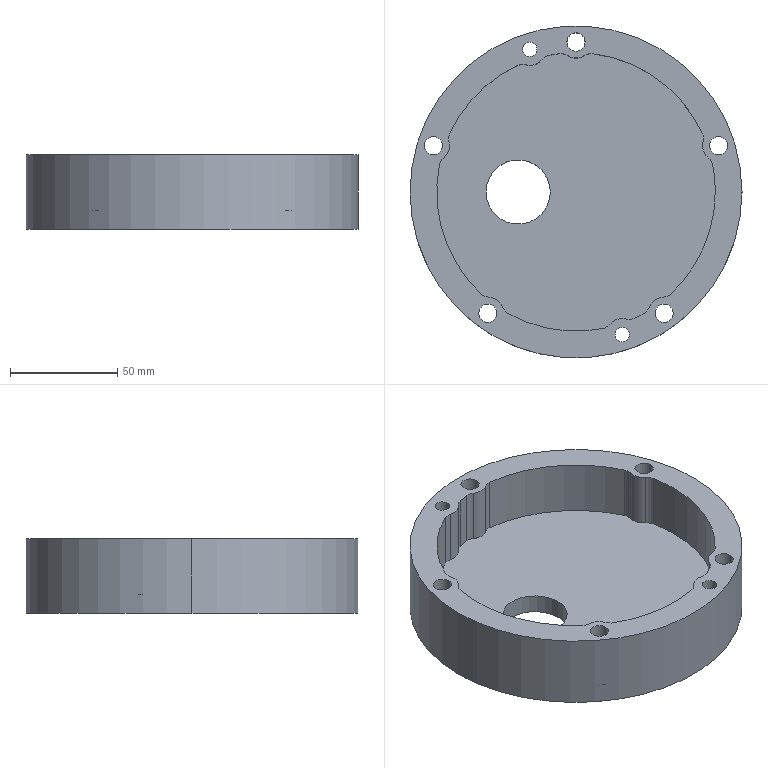Component | SolidWorks | 8RearFlange-1 | 1 solid | 67 faces | box 155 x 155 x 35 mm | volume 295651 mm3 | cylinder 59 | plane 8 | commonest cylinder face diameters 10 x15 14 x10 8.5 x10 130 x8 15 x8 6.8 x4 155 x2 30 x2
build123d program:
from build123d import *

# Parameters (mm, degrees)
SKETCH68_R           = 77.5
BOSS_EXTRUDE10_DEPTH = 35
SKETCH69_R           = 4.25
CUT_EXTRUDE20_DEPTH  = 116.054
SKETCH71_R           = 7
CUT_EXTRUDE21_DEPTH  = 9
CIRPATTERN7_COUNT    = 5
SKETCH72_R           = 15
CUT_EXTRUDE22_DEPTH  = 116.054
M8_TAPPED_HOLE1_D    = 6.8
CIRPATTERN8_COUNT    = 2
CUT_EXTRUDE23_DEPTH  = 26
FILLET1_R            = 5


with BuildPart() as part:
    # Sketch68 → Boss-Extrude10 (new body)
    with BuildSketch(Plane.XY):
        Circle(SKETCH68_R)
    extrude(amount=BOSS_EXTRUDE10_DEPTH)

    # Sketch69 → Cut-Extrude20 (cut, through all)
    with BuildSketch(Plane.XY.offset(35)):
        with Locations((0, 70)):
            Circle(SKETCH69_R)
    cut_extrude20 = extrude(amount=-CUT_EXTRUDE20_DEPTH, mode=Mode.SUBTRACT)

    # Sketch71 → Cut-Extrude21 (cut)
    with BuildSketch(Plane(origin=(0, 0, 0), x_dir=(-1, 0, 0), z_dir=(0, 0, -1))):
        with Locations((0, 70)):
            Circle(SKETCH71_R)
    cut_extrude21 = extrude(amount=-CUT_EXTRUDE21_DEPTH, mode=Mode.SUBTRACT)

    # CirPattern7: Cut-Extrude20, Cut-Extrude21 ×5 about axis
    cirpattern7_axis = Axis((0, 0, 0), (0, 0, 1))
    add([cut_extrude20.rotate(cirpattern7_axis, i * 360 / CIRPATTERN7_COUNT) for i in range(1, CIRPATTERN7_COUNT)], mode=Mode.SUBTRACT)
    add([cut_extrude21.rotate(cirpattern7_axis, i * 360 / CIRPATTERN7_COUNT) for i in range(1, CIRPATTERN7_COUNT)], mode=Mode.SUBTRACT)

    # Sketch72 → Cut-Extrude22 (cut, through all)
    with BuildSketch(Plane.XY.offset(35)):
        with Locations((-27, 0)):
            Circle(SKETCH72_R)
    extrude(amount=-CUT_EXTRUDE22_DEPTH, mode=Mode.SUBTRACT)

    # M8 Tapped Hole1 (through all)
    with Locations(Plane.XY.offset(35)):
        with Locations((-21.631, 66.574)):
            m8_tapped_hole1 = Hole(M8_TAPPED_HOLE1_D / 2)

    # CirPattern8: M8 Tapped Hole1 ×2 about axis
    cirpattern8_axis = Axis((0, 0, 0), (0, 0, 1))
    for i in range(1, CIRPATTERN8_COUNT):
        add(m8_tapped_hole1.rotate(cirpattern8_axis, i * 360 / CIRPATTERN8_COUNT), mode=Mode.SUBTRACT)

    # Sketch76 → Cut-Extrude23 (cut)
    with BuildSketch(Plane.XY.offset(35)):
        with BuildLine():
            ThreePointArc((42.429, -49.242), (59.088, -27.084), (65, 0))
            ThreePointArc((65, 0), (64.566, 7.499), (63.27, 14.898))
            ThreePointArc((63.27, 14.898), (59.441, 19.314), (59.943, 25.136))
            ThreePointArc((59.943, 25.136), (38.206, 52.586), (5.382, 64.777))
            ThreePointArc((5.382, 64.777), (0, 62.5), (-5.382, 64.777))
            ThreePointArc((-5.382, 64.777), (-10.168, 64.2), (-14.898, 63.27))
            ThreePointArc((-14.898, 63.27), (-19.314, 59.441), (-25.136, 59.943))
            ThreePointArc((-25.136, 59.943), (-45.962, 45.962), (-59.943, 25.136))
            ThreePointArc((-59.943, 25.136), (-59.295, 23.437), (-59.074, 21.631))
            ThreePointArc((-59.074, 21.631), (-60.209, 17.665), (-63.27, 14.898))
            ThreePointArc((-63.27, 14.898), (-61.819, -20.086), (-42.429, -49.242))
            ThreePointArc((-42.429, -49.242), (-36.737, -50.564), (-33.721, -55.569))
            ThreePointArc((-33.721, -55.569), (-10.168, -64.2), (14.898, -63.27))
            ThreePointArc((14.898, -63.27), (19.314, -59.441), (25.136, -59.943))
            ThreePointArc((25.136, -59.943), (29.509, -57.915), (33.721, -55.569))
            ThreePointArc((33.721, -55.569), (36.737, -50.564), (42.429, -49.242))
        make_face()
    extrude(amount=-CUT_EXTRUDE23_DEPTH, mode=Mode.SUBTRACT)

    # Fillet1
    fillet1_edges = [part.edges().sort_by_distance(p)[0] for p in [
        (42.429, -49.242, 22),
        (33.721, -55.569, 22),
        (25.136, -59.943, 22),
        (14.898, -63.27, 22),
        (-33.721, -55.569, 22),
        (-42.429, -49.242, 22),
        (-63.27, 14.898, 22),
        (-59.943, 25.136, 22),
        (-25.136, 59.943, 22),
        (-14.898, 63.27, 22),
        (-5.382, 64.777, 22),
        (5.382, 64.777, 22),
        (59.943, 25.136, 22),
        (63.27, 14.898, 22),
    ]]
    fillet(fillet1_edges, radius=FILLET1_R)


solid = part.part

# Placed as in the assembly
solid = solid.moved(Location((33.957, 1.776, 135), (0, 0, 0)))